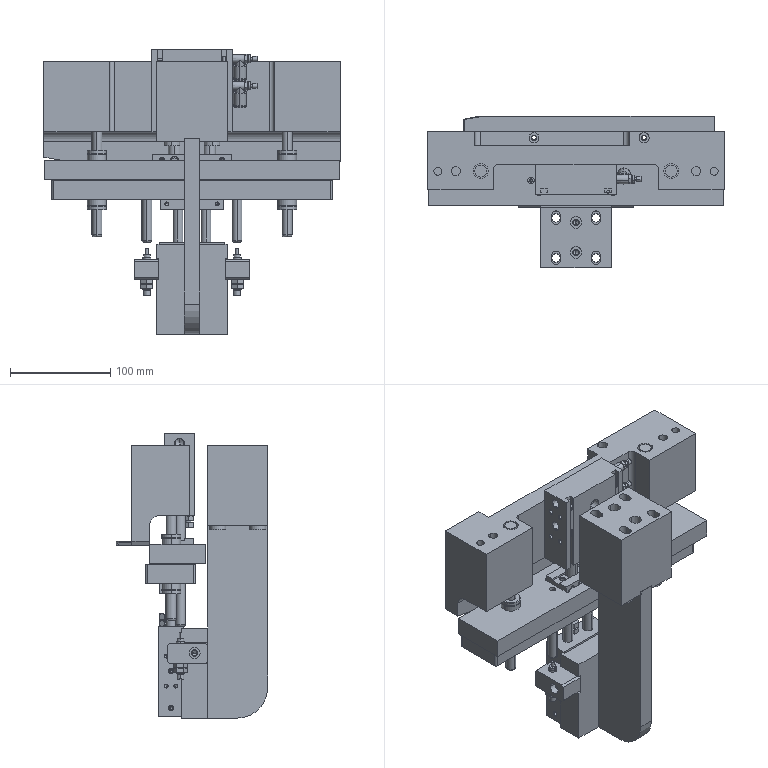Assembly | SolidWorks | mm | 32 component files | 32 solids | 1253 faces | box 296 x 151.72 x 283.93 mm | volume 2520689 mm3 | plane 499 | cylinder 483 | cone 244 | torus 24 | sphere 2 | spline 1 | commonest cylinder face diameters 10 x42 4.134 x36 11 x28 5 x24 8 x24 19 x24 3.242 x24 8.5 x20
Bill of materials:
2SZT-0-004 | 1 |  | Rectangular prismatic block with a pattern of slots and holes through the top face and a small notch at the bottom of one side.
2SZT-0-009 | 1 |  | Long thin flat strip with four small holes in a row and one angled or tapered end.
2SZT-2-001 | 1 |  | Rectangular bar with slightly rounded vertical corners and a symmetric row of through holes in three sizes.
2SZT-2-002-2 | 1 |  | Long block with taller end pads, a long central recess or cutout, and a stepped L-shaped cross-section with a large inside fillet.
2SZT-2-003 | 2 |  | Slender cylindrical pin with a short, slightly larger diameter head at one end and a slightly rounded opposite end.
2SZT-2-005 | 1 |  | Bracket-like body: a tall rectangular plate with one large rounded corner, joined to a shorter side block with notches and a small side hole.
2SZT-2-006 | 1 |  | Rectangular bar with two large through holes near the ends, four small center holes, and a shallow narrow groove pattern on the top face.
2SZT-2-007 | 2 |  | Rectangular block with chamfered long edges and two perpendicular round holes.
2SZT-2-010 | 2 |  | Solid cylindrical rod with a small axial hole in one end face and a rounded or chamfered edge at the other end.
AS1201_M5_F04 | 2 |  | T-shaped body made of turned sections. A horizontal stepped cylindrical body is joined at a right angle to a larger vertical cylindrical body. The horizontal body has a chamfered small-diameter stub at one end, a main cylinder, then a hex-like flat section, a collar, a reduced-diameter neck and a cylindrical end spigot. The vertical body has a smaller neck that widens into a larger cylinder, with a groove and a flange-like lip near its bottom end.
LMU_N10 | 4 |  | Hollow cylindrical sleeve with a concentric through-bore. It has two shallow circumferential grooves, one near each end, and small edge chamfers or rounds on both ends.
Part1342542 | 4 |  | Flat annular ring (washer-like): a plain cylindrical outer and inner diameter with flat faces.
RB0806 | 2 |  | Stepped cylindrical body with two hexagonal collars near one end, a small protruding pin at the other end, and a small notch at the base end.
Mates:
1. coincident | RB0806-2 face at (1003.63, 378.593, -409.597) dir (-0.00002551, 0, -1) | RB0806-3 face at (913.63, 378.593, -409.595) dir (-0.00002551, 0, -1)
2. concentric | 2SZT-2-007-2 face at (1000.264, 375.193, -373.197) dir (0.00002551, 0, 1) r 4 | RB0806-2 face at (1000.263, 375.193, -393.197) dir (0.00002551, 0, 1) r 4
3. coincident | 2SZT-2-007-2 face at (1012.263, 388.093, -393.197) dir (-0.00002551, 0, -1) | 2SZT-2-007-5 face at (898.263, 388.093, -393.194) dir (-0.00002551, 0, -1)
4. concentric | RB0806-3 face at (910.263, 375.193, -393.195) dir (0.00002551, 0, 1) r 4 | 2SZT-2-007-5 edge at (910.263, 375.193, -393.195) dir (-0.00002551, 0, -1) r 4
5. concentric | LMU_N10-8 face at (860.266, 384.385, -264.262) dir (-0.00002551, 0, -1) r 9.5 | 2SZT-2-006-3 face at (860.266, 384.385, -274.262) dir (-0.00002551, 0, -1) r 9.51
6. coincident | 2SZT-2-006-3 face at (807.766, 350.193, -293.261) dir (-0.00002551, 0, -1) | LMU_N10-8 face at (860.266, 393.485, -293.262) dir (-0.00002551, 0, -1)
7. concentric | 2SZT-2-006-3 face at (1050.266, 384.385, -274.267) dir (-0.00002551, 0, -1) r 9.51 | LMU_N10-7 face at (1050.266, 384.385, -264.267) dir (-0.00002551, 0, -1) r 9.5
8. coincident | 2SZT-2-006-3 face at (807.766, 350.193, -293.261) dir (-0.00002551, 0, -1) | LMU_N10-7 face at (1050.266, 393.485, -293.267) dir (-0.00002551, 0, -1)
9. coincident | 2SZT-2-005-1 face at (922.263, 374.093, -393.22) dir (-1, 0, 0.00002551) | 2SZT-2-007-5 face at (922.263, 388.093, -393.195) dir (1, 0, -0.00002551)
10. coincident | 2SZT-2-005-1 face at (988.263, 374.093, -393.222) dir (1, 0, -0.00002551) | 2SZT-2-007-2 face at (988.264, 388.093, -373.197) dir (-1, 0, 0.00002551)
11. concentric | 2SZT-2-001-3 face at (1050.266, 384.385, -295.198) dir (0.00002551, 0, 1) r 9.51 | LMU_N10-9 face at (1050.266, 384.385, -295.198) dir (-0.00002551, 0, -1) r 9.5
12. concentric | 2SZT-2-001-3 face at (860.266, 384.385, -295.193) dir (0.00002551, 0, 1) r 9.51 | LMU_N10-10 face at (860.266, 384.385, -295.193) dir (-0.00002551, 0, -1) r 9.5
13. coincident | 2SZT-2-001-3 face at (1095.266, 360.093, -295.199) dir (0.00002551, 0, 1) | LMU_N10-9 face at (1050.266, 389.385, -295.198) dir (0.00002551, 0, 1)
14. coincident | 2SZT-2-001-3 face at (1095.266, 360.093, -295.199) dir (0.00002551, 0, 1) | LMU_N10-10 face at (860.266, 389.385, -295.193) dir (0.00002551, 0, 1)
15. concentric | 2SZT-2-002-2-1 face at (1050.269, 384.385, -175.948) dir (-0.00002551, 0, -1) r 5.01 | 2SZT-2-003-5 face at (1050.264, 384.385, -350.948) dir (0.00002551, 0, 1) r 5
16. coincident | 2SZT-2-002-2-1 face at (1103.269, 402.155, -175.95) dir (0.00002551, 0, 1) | 2SZT-2-003-5 face at (1050.269, 384.385, -175.948) dir (0.00002551, 0, 1)
17. concentric | 2SZT-2-002-2-1 face at (860.269, 384.385, -175.943) dir (-0.00002551, 0, -1) r 5.01 | 2SZT-2-003-6 face at (860.264, 384.385, -350.943) dir (0.00002551, 0, 1) r 5
18. coincident | 2SZT-2-002-2-1 face at (1103.269, 402.155, -175.95) dir (0.00002551, 0, 1) | 2SZT-2-003-6 face at (860.269, 384.385, -175.943) dir (0.00002551, 0, 1)
19. concentric | 2SZT-2-005-1 face at (988.263, 361.093, -383.197) dir (1, 0, -0.00002551) r 2.5 | 2SZT-2-007-2 face at (1012.263, 361.093, -383.197) dir (1, 0, -0.00002551) r 3.3
20. parallel | 2SZT-2-005-1 face at (920.264, 374.093, -358.195) dir (0.00002551, 0, 1) | 2SZT-2-007-2 face at (1012.264, 388.093, -373.197) dir (0.00002551, 0, 1)
21. concentric | 2SZT-2-005-1 face at (922.263, 361.093, -383.195) dir (-1, 0, 0.00002551) r 2.5 | 2SZT-2-007-5 face at (898.263, 361.093, -383.194) dir (-1, 0, 0.00002551) r 3.3
22. concentric | LMU_N10-10 face at (860.266, 384.385, -295.193) dir (-0.00002551, 0, -1) r 5 | 2SZT-2-003-6 face at (860.264, 384.385, -350.943) dir (0.00002551, 0, 1) r 5
23. coincident | 2SZT-2-002-2-1 face at (1103.266, 424.655, -271.5) dir (-0.00002551, 0, -1) | 2SZT-0-009-3 face at (1093.266, 410.465, -271.499) dir (0.00002551, 0, 1)
24. concentric | 2SZT-2-002-2-1 face at (883.266, 417.715, -271.494) dir (-0.00002551, 0, -1) r 2.005 | 2SZT-0-009-3 face at (883.266, 417.715, -271.494) dir (0.00002551, 0, 1) r 2.005
25. concentric | 2SZT-2-002-2-1 face at (1053.266, 417.715, -271.498) dir (-0.00002551, 0, -1) r 2.005 | 2SZT-0-009-3 face at (1053.266, 417.715, -271.498) dir (0.00002551, 0, 1) r 2.005
26. concentric | LMU_N10-9 face at (1050.266, 384.385, -295.198) dir (-0.00002551, 0, -1) r 5 | 2SZT-2-003-5 face at (1050.264, 384.385, -350.948) dir (0.00002551, 0, 1) r 5
27. concentric | 2SZT-2-005-1 face at (955.262, 372.093, -416.196) dir (0, 1, 0) r 2.5 | CXSM20-20-Z73(0_0_0)-1/CXSM20-20(0_0)_BODY-1 edge at (955.262, 372.093, -416.196) dir (0, -1, 0) r 3
28. concentric | 2SZT-2-005-1 face at (955.263, 372.093, -386.196) dir (0, 1, 0) r 2.5 | CXSM20-20-Z73(0_0_0)-1/CXSM20-20(0_0)_BODY-1 edge at (955.263, 397.093, -386.196) dir (0, -1, 0) r 4.75
29. coincident | 2SZT-2-005-1 face at (923.265, 372.093, -321.411) dir (0, 1, 0) | CXSM20-20-Z73(0_0_0)-1/CXSM20-20(0_0)_BODY-1 face at (923.262, 372.093, -446.195) dir (0, -1, 0)
30. coincident | 2SZT-2-001-3 face at (924.265, 396.093, -312.195) dir (-0.00002551, 0, -1) | CXSM20-20-Z73(0_0_0)-1/CXSM20-20(0_0)_ROD-1 face at (955.265, 384.593, -312.196) dir (0.00002551, 0, 1)
31. concentric | 2SZT-2-001-3 face at (930.266, 384.593, -295.195) dir (0.00002551, 0, 1) r 2.75 | CXSM20-20-Z73(0_0_0)-1/CXSM20-20(0_0)_ROD-1 face at (930.265, 384.593, -322.195) dir (0.00002551, 0, 1) r 2.067
32. concentric | 2SZT-2-001-3 face at (980.266, 384.593, -295.197) dir (0.00002551, 0, 1) r 2.75 | CXSM20-20-Z73(0_0_0)-1/CXSM20-20(0_0)_ROD-1 face at (980.265, 384.593, -322.197) dir (0.00002551, 0, 1) r 2.067
33. coincident | 2SZT-2-006-3 face at (1000.266, 375.193, -286.266) dir (-0.00002551, 0, -1) | 2SZT-2-010-1 face at (1000.266, 375.193, -286.266) dir (0.00002551, 0, 1)
34. concentric | 2SZT-2-006-3 face at (1000.266, 375.193, -286.266) dir (-0.00002551, 0, -1) r 5 | 2SZT-2-010-1 face at (1000.264, 375.193, -356.266) dir (0.00002551, 0, 1) r 5
35. coincident | 2SZT-2-006-3 face at (925.266, 379.443, -286.464) dir (-0.00002551, 0, -1) | 2SZT-2-010-2 face at (910.266, 375.193, -286.464) dir (0.00002551, 0, 1)
36. concentric | 2SZT-2-006-3 face at (910.266, 375.193, -286.264) dir (-0.00002551, 0, -1) r 5 | 2SZT-2-010-2 face at (910.264, 375.193, -356.464) dir (0.00002551, 0, 1) r 5
37. concentric | 2SZT-2-005-1 face at (955.267, 333.093, -252.696) dir (0.00002551, 0, 1) r 3 | 2SZT-0-004-1 face at (955.269, 333.093, -175.946) dir (0.00002551, 0, 1) r 3.25
38. concentric | 2SZT-2-005-1 face at (955.267, 303.093, -252.696) dir (0.00002551, 0, 1) r 3 | 2SZT-0-004-1 face at (955.269, 303.093, -175.946) dir (0.00002551, 0, 1) r 3.25
39. coincident | 2SZT-2-005-1 face at (962.767, 288.093, -252.696) dir (0.00002551, 0, 1) | 2SZT-0-004-1 face at (962.767, 416.28, -252.696) dir (-0.00002551, 0, -1)
40. coincident | 2SZT-2-002-2-1 face at (1103.269, 402.155, -175.95) dir (0.00002551, 0, 1) | 2SZT-0-004-1 face at (920.269, 287.75, -175.945) dir (0.00002551, 0, 1)
41. coincident | 2SZT-0-004-1 axis at (935.269, 297.75, -175.945) dir (-0.00002551, 0, -1) | Part1342542-1 axis at (935.266, 297.75, -259.945) dir (0.00002551, 0, 1)
42. coincident | 2SZT-0-004-1 axis at (935.269, 337.75, -175.945) dir (-0.00002551, 0, -1) | Part1342542-2 axis at (935.266, 337.75, -259.945) dir (0.00002551, 0, 1)
43. coincident | 2SZT-0-004-1 axis at (975.269, 297.75, -175.946) dir (-0.00002551, 0, -1) | Part1342542-3 axis at (975.266, 297.75, -259.946) dir (0.00002551, 0, 1)
44. coincident | 2SZT-0-004-1 axis at (975.269, 337.75, -175.946) dir (-0.00002551, 0, -1) | Part1342542-4 axis at (975.266, 337.75, -259.946) dir (0.00002551, 0, 1)
45. coincident | 2SZT-0-004-1 face at (920.267, 287.75, -255.945) dir (-0.00002551, 0, -1) | Part1342542-3 face at (975.267, 297.75, -255.946) dir (0.00002551, 0, 1)
46. coincident | 2SZT-0-004-1 face at (920.267, 287.75, -255.945) dir (-0.00002551, 0, -1) | Part1342542-4 face at (975.267, 337.75, -255.946) dir (0.00002551, 0, 1)
47. coincident | 2SZT-0-004-1 face at (920.267, 287.75, -255.945) dir (-0.00002551, 0, -1) | Part1342542-2 face at (935.267, 337.75, -255.945) dir (0.00002551, 0, 1)
48. coincident | 2SZT-0-004-1 face at (920.267, 287.75, -255.945) dir (-0.00002551, 0, -1) | Part1342542-1 face at (935.267, 297.75, -255.945) dir (0.00002551, 0, 1)
49. concentric | AS1201_M5_F04-6 face at (1007.768, 376.143, -200.266) dir (-1, 0, 0.00002551) r 2.5 | CXSM25-10-Z73(0_0_0)-2/CXSM25-10(0_0)_BODY-1 face at (986.295, 376.143, -200.266) dir (1, 0, -0.00002551) r 4.283
50. concentric | AS1201_M5_F04-5 face at (1007.769, 376.143, -173.266) dir (-1, 0, 0.00002551) r 4.5 | CXSM25-10-Z73(0_0_0)-2/CXSM25-10(0_0)_BODY-1 face at (986.296, 376.143, -173.266) dir (1, 0, -0.00002551) r 4.283
51. coincident | AS1201_M5_F04-5 face at (995.269, 376.627, -175.216) dir (-1, 0, 0.00002551) | CXSM25-10-Z73(0_0_0)-2/CXSM25-10(0_0)_BODY-1 face at (995.269, 391.143, -164.266) dir (1, 0, -0.00002551)
52. coincident | AS1201_M5_F04-6 face at (995.268, 376.627, -202.216) dir (-1, 0, 0.00002551) | CXSM25-10-Z73(0_0_0)-2/CXSM25-10(0_0)_BODY-1 face at (995.269, 391.143, -164.266) dir (1, 0, -0.00002551)
53. concentric | 2SZT-2-006-3 face at (985.266, 376.143, -293.266) dir (-0.00002551, 0, -1) r 3.3 | CXSM25-10-Z73(0_0_0)-2/CXSM25-10(0_0)_ROD-1 face at (985.266, 376.143, -270.266) dir (-0.00002551, 0, -1) r 2.458
54. concentric | 2SZT-2-006-3 face at (925.266, 376.143, -293.264) dir (-0.00002551, 0, -1) r 3.3 | CXSM25-10-Z73(0_0_0)-2/CXSM25-10(0_0)_ROD-1 face at (925.266, 376.143, -270.264) dir (-0.00002551, 0, -1) r 2.458
55. coincident | 2SZT-2-006-3 face at (1102.766, 350.193, -280.269) dir (0.00002551, 0, 1) | CXSM25-10-Z73(0_0_0)-2/CXSM25-10(0_0)_ROD-1 face at (955.266, 376.143, -280.265) dir (-0.00002551, 0, -1)
56. concentric | LMU_N10-7 face at (1050.266, 384.385, -264.267) dir (-0.00002551, 0, -1) r 5 | 2SZT-2-003-5 face at (1050.264, 384.385, -350.948) dir (0.00002551, 0, 1) r 5
57. concentric | LMU_N10-8 face at (860.266, 384.385, -264.262) dir (-0.00002551, 0, -1) r 5 | 2SZT-2-003-6 face at (860.264, 384.385, -350.943) dir (0.00002551, 0, 1) r 5
58. concentric | 2SZT-2-002-2-1 face at (955.268, 409.655, -216.265) dir (0, 1, 0) r 4.5 | CXSM25-10-Z73(0_0_0)-2/CXSM25-10(0_0)_BODY-1 face at (955.268, 361.143, -216.265) dir (0, 1, 0) r 3.45
59. coincident | 2SZT-2-007-2 face at (1012.263, 388.093, -393.197) dir (-0.00002551, 0, -1) | RB0806-3 face at (910.263, 375.193, -393.195) dir (0.00002551, 0, 1)
60. coincident | CXSM20-20(0_0)_BODY-1 axis at (-80.9, 0, 0) dir (1, 0, 0) | CXSM20-20(0_0)_ROD-1 axis at (60.9, 0, 0) dir (-1, 0, 0)
61. angle | CXSM20-20(0_0)_ROD-1 plane at (-20, 0, 0) dir (0, 0, 1) | CXSM20-20(0_0)_BODY-1 plane at (0, 0, 0) dir (0, 0, 1)
62. coincident | CXSM20-20(0_0)_BODY-1 axis at (80.9, -26.5, 7.1) dir (-1, 0, 0) | CXS_D-Z73-1 axis at (-42.9, -26.5, 7.1) dir (1, 0, 0)
63. distance | CXS_D-Z73-2 plane at (83, 26.5, 7.1) dir (-1, 0, 0) | CXSM20-20(0_0)_BODY-1 plane at (90, 0, 0) dir (1, 0, 0)
64. coincident | CXSM20-20(0_0)_BODY-1 axis at (80.9, 26.5, 7.1) dir (-1, 0, 0) | CXS_D-Z73-2 axis at (2.1, 26.5, 7.1) dir (1, 0, 0)
65. angle | CXS_D-Z73-2 plane at (83, 26.5, 7.1) dir (0, 1, 0) | CXSM20-20(0_0)_BODY-1 plane at (0, 0, 7.1) dir (0, 0, 1)
66. distance | CXSM20-20(0_0)_BODY-1 face at (-12, 0, 6.5) dir (-1, 0, 0) | CXSM20-20(0_0)_ROD-1 face at (-32, 0, 0) dir (1, 0, 0)
67. coincident | CXSM25-10(0_0)_BODY-1 axis at (-80.9, 0, 0) dir (1, 0, 0) | CXSM25-10(0_0)_ROD-1 axis at (70.9, 0, 0) dir (-1, 0, 0)
68. angle | CXSM25-10(0_0)_ROD-1 plane at (-10, 0, 0) dir (0, 0, 1) | CXSM25-10(0_0)_BODY-1 plane at (0, 0, 0) dir (0, 0, 1)
69. coincident | CXSM25-10(0_0)_BODY-1 axis at (80.9, -32, 9.6) dir (-1, 0, 0) | CXS_D-Z73-1 axis at (-42.9, -32, 9.6) dir (1, 0, 0)
70. distance | CXS_D-Z73-2 plane at (73, 32, 9.6) dir (-1, 0, 0) | CXSM25-10(0_0)_BODY-1 plane at (82, 0, 0) dir (1, 0, 0)
71. coincident | CXSM25-10(0_0)_BODY-1 axis at (80.9, 32, 9.6) dir (-1, 0, 0) | CXS_D-Z73-2 axis at (-7.9, 32, 9.6) dir (1, 0, 0)
72. angle | CXS_D-Z73-2 plane at (73, 32, 9.6) dir (0, 1, 0) | CXSM25-10(0_0)_BODY-1 plane at (0, 0, 9.6) dir (0, 0, 1)
73. distance | CXSM25-10(0_0)_BODY-1 face at (-12, 0, 9) dir (-1, 0, 0) | CXSM25-10(0_0)_ROD-1 face at (-22, 0, 0) dir (1, 0, 0)